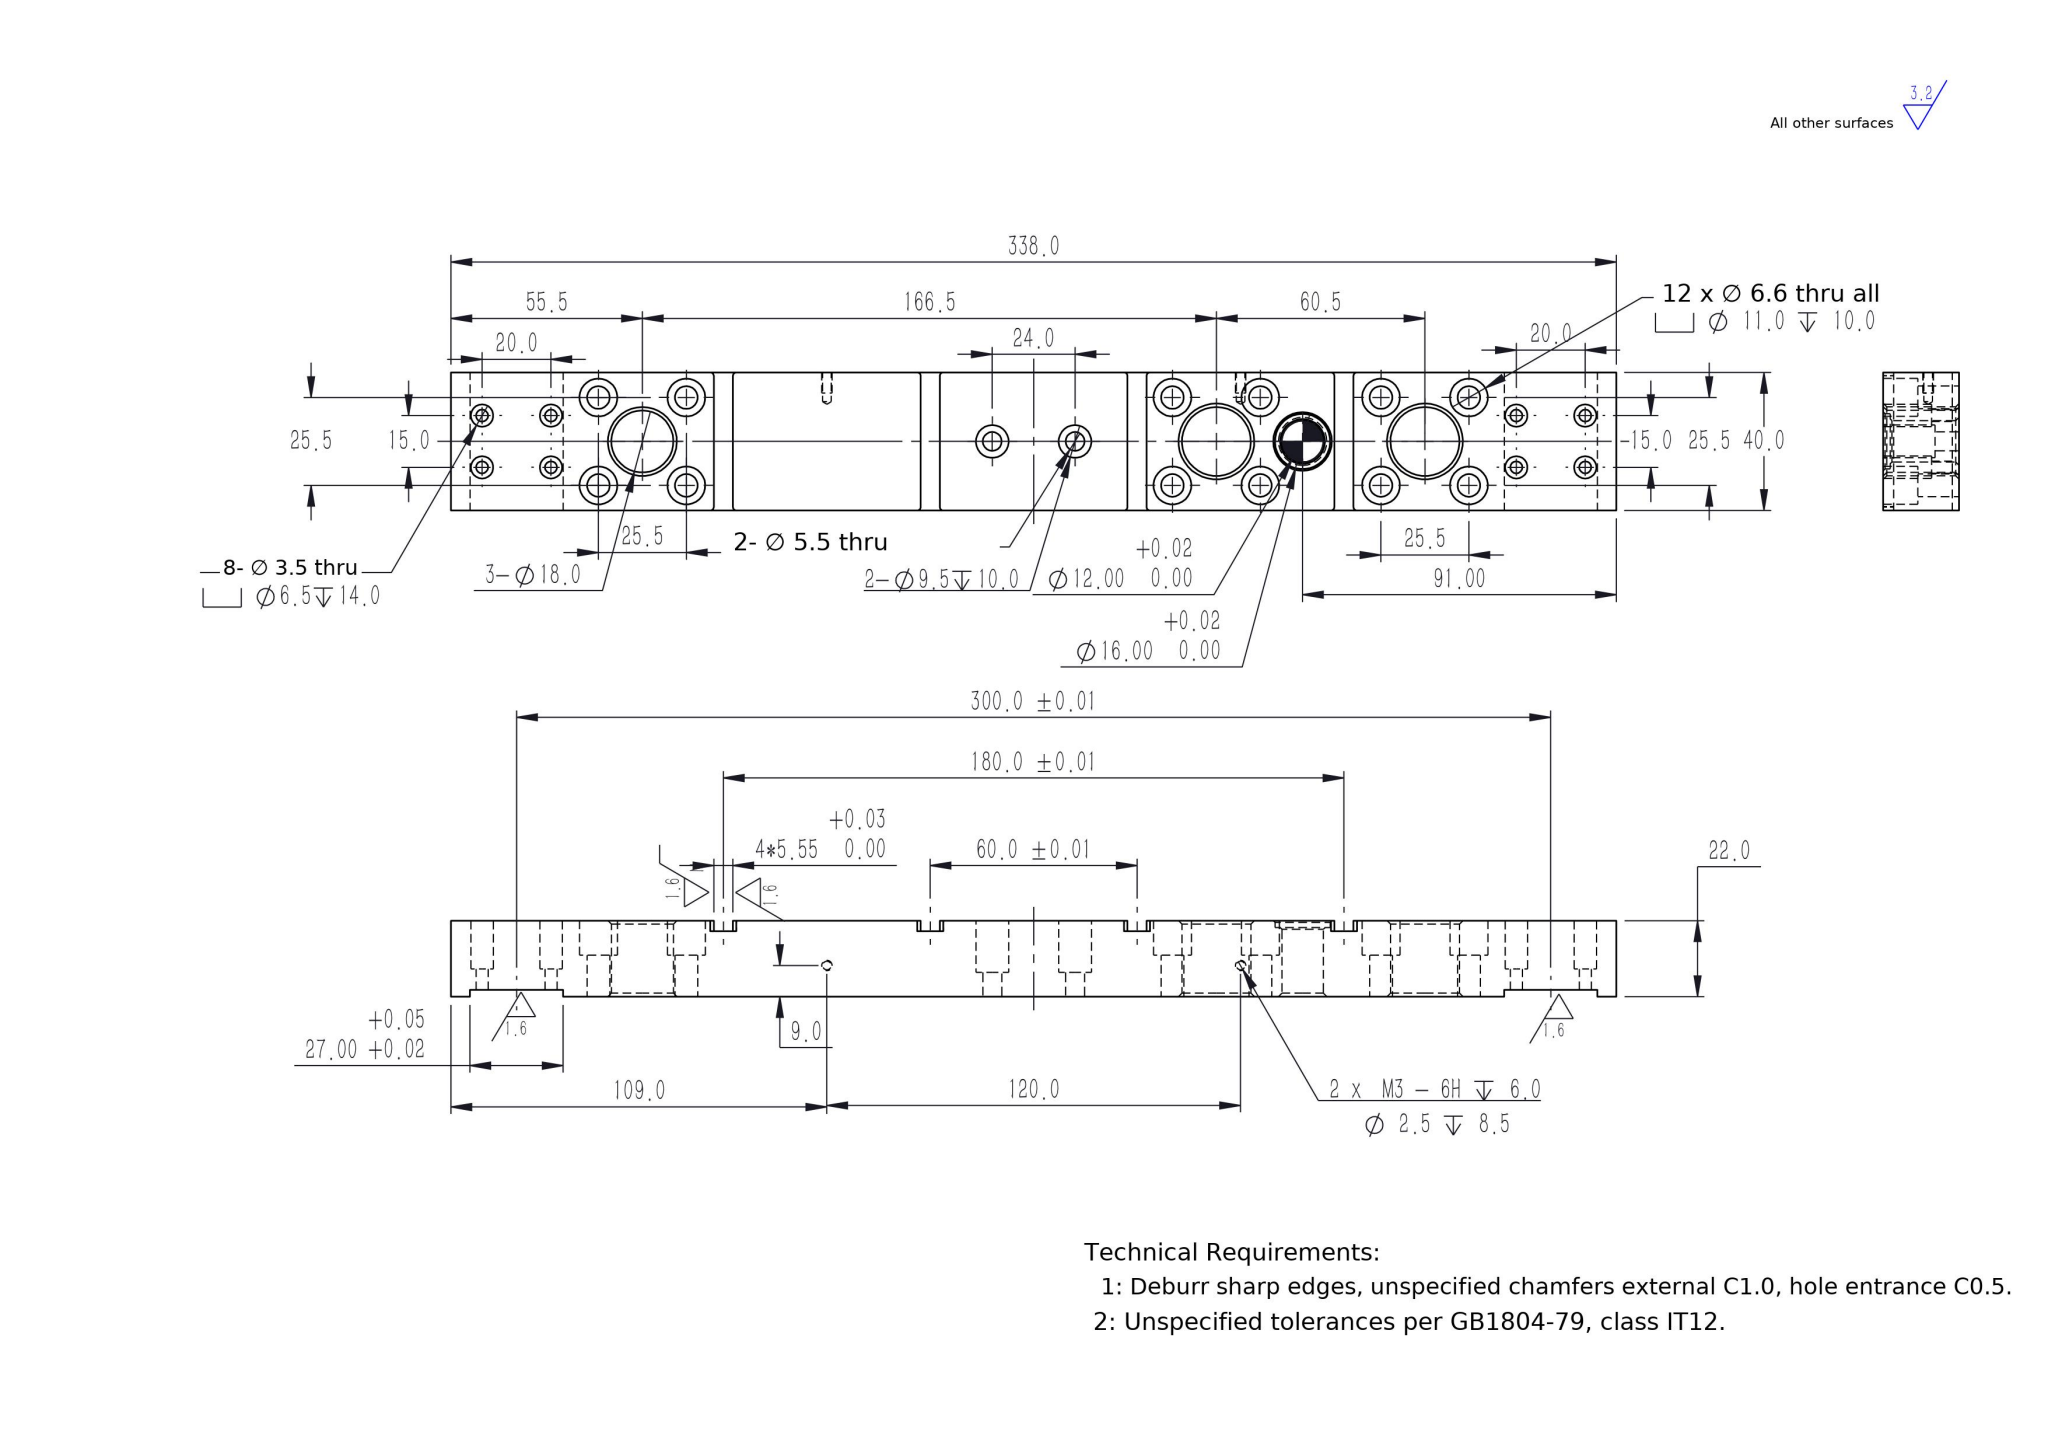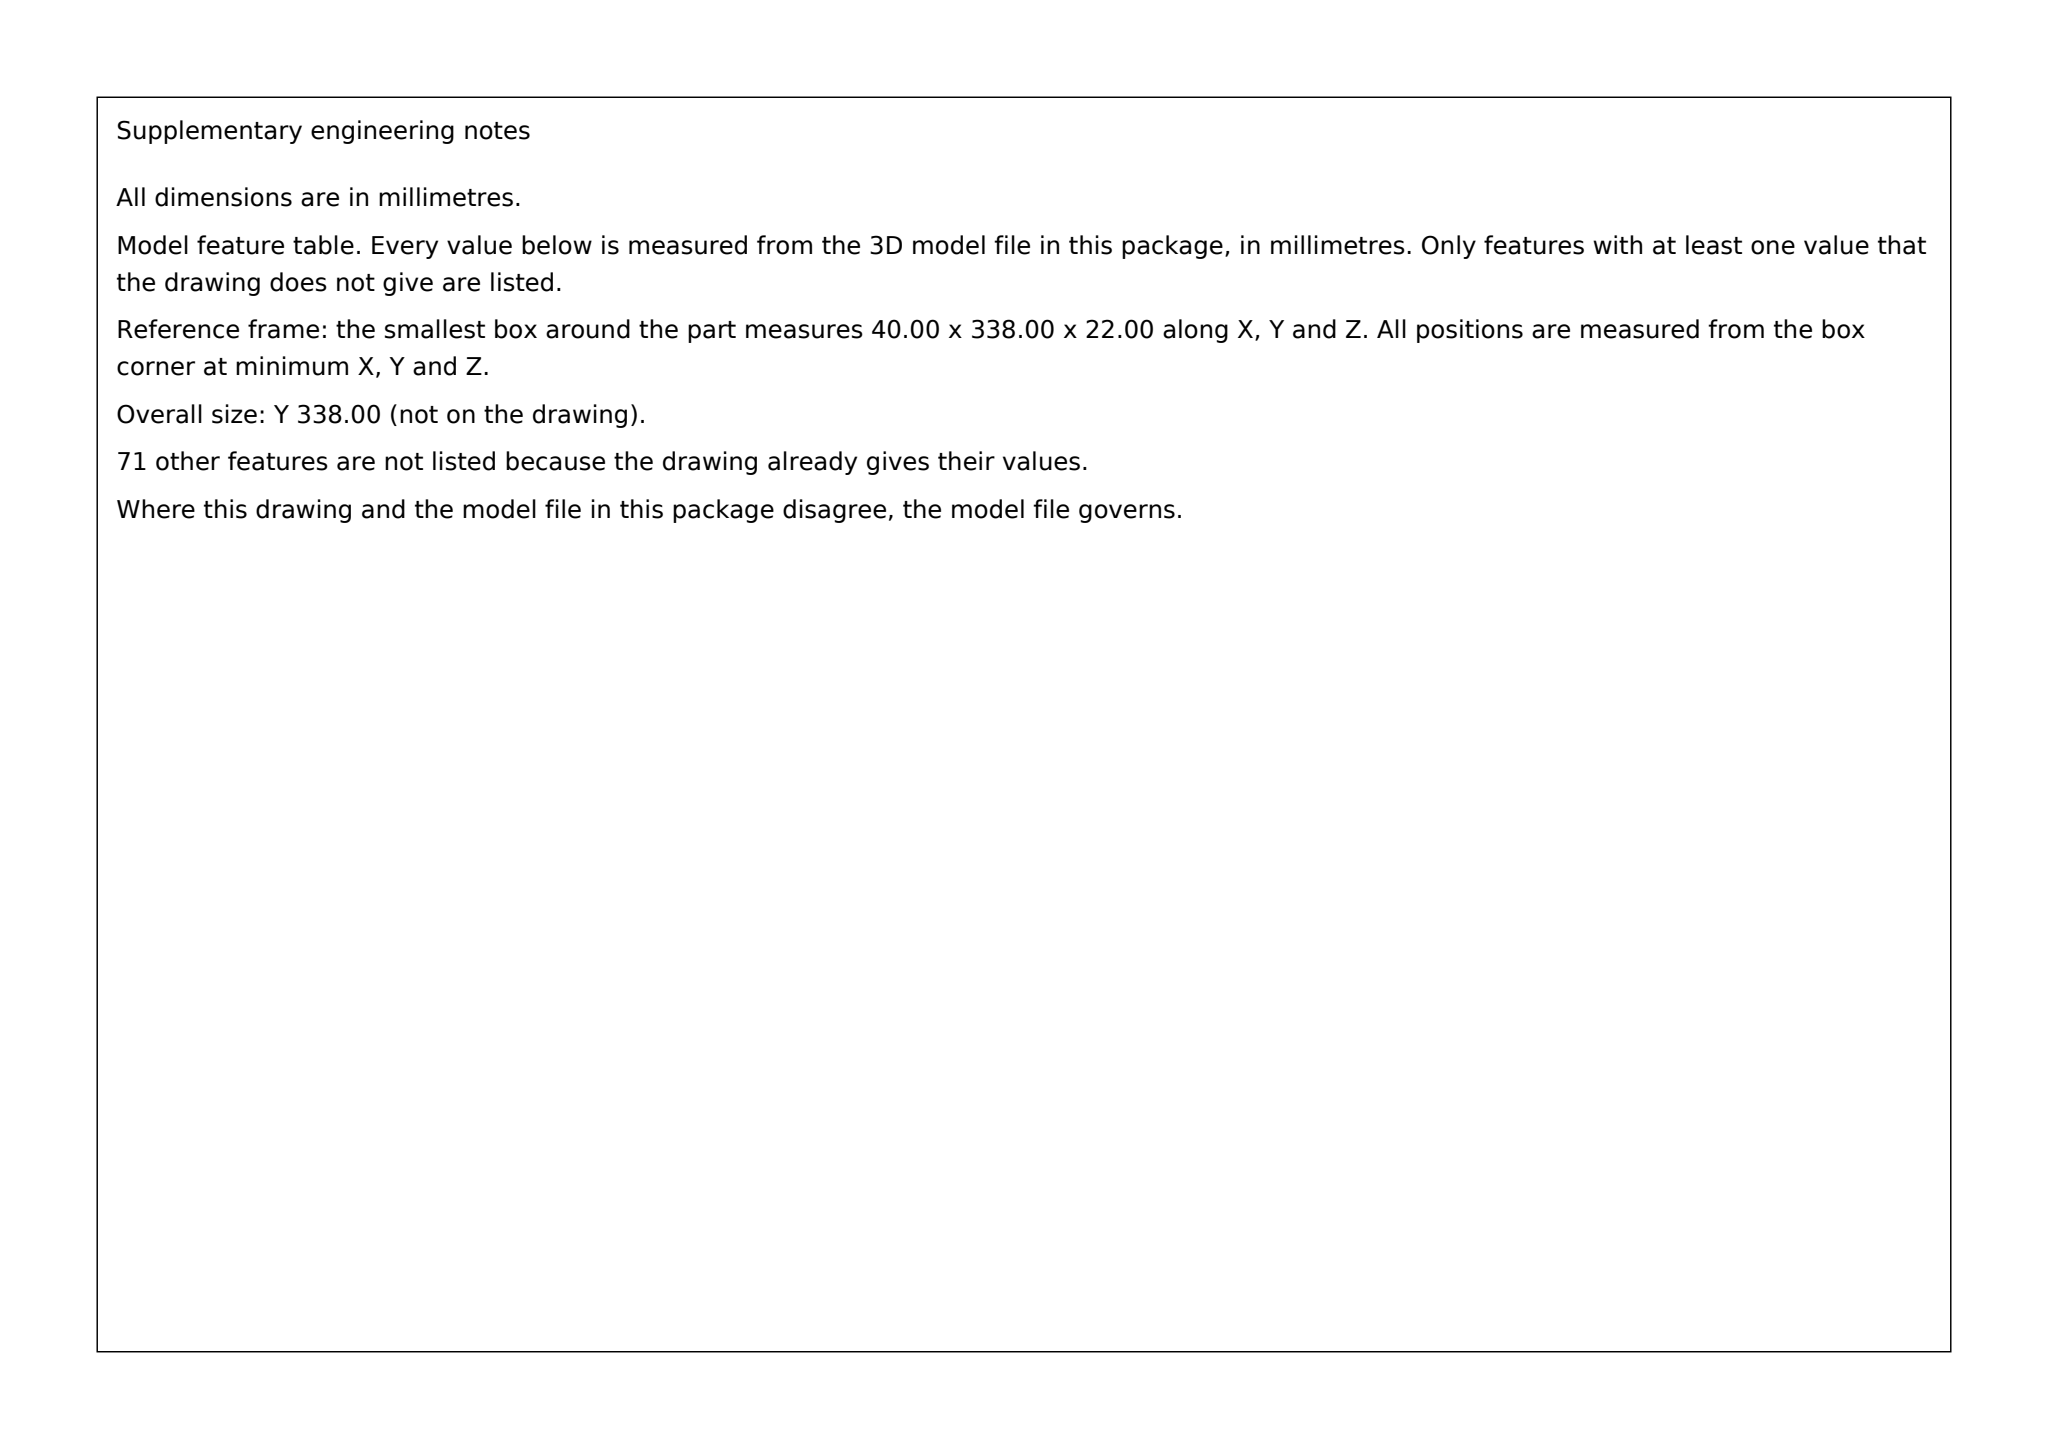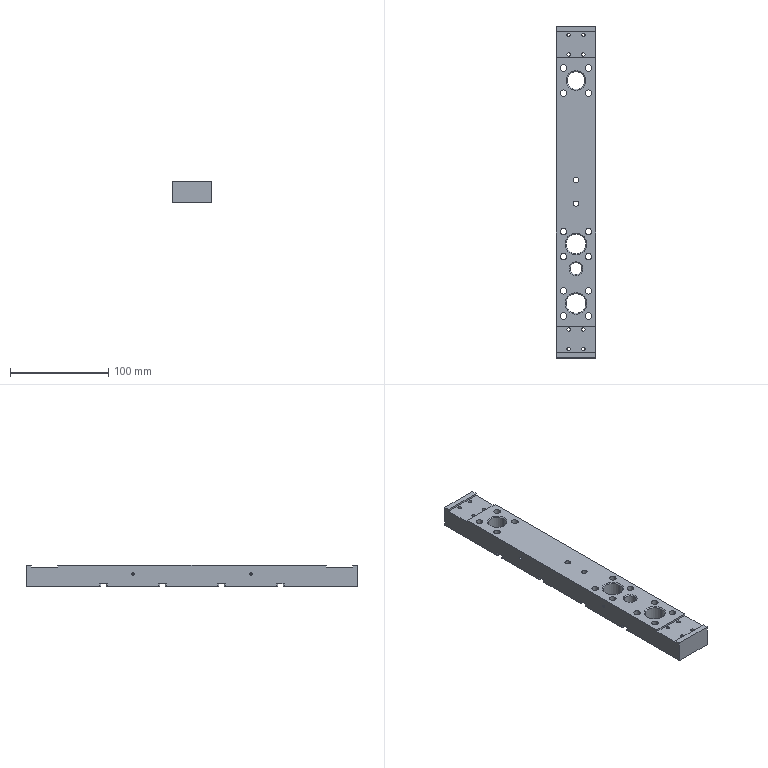Part | SolidWorks | mm | 1 solid | 193 faces | box 40 x 338 x 22 mm | volume 245087 mm3 | cylinder 118 | plane 53 | cone 22 | commonest cylinder face diameters 11 x24 6.6 x24 6.5 x16 3.5 x16 2 x16 2.5 x4 20 x4 9.5 x4